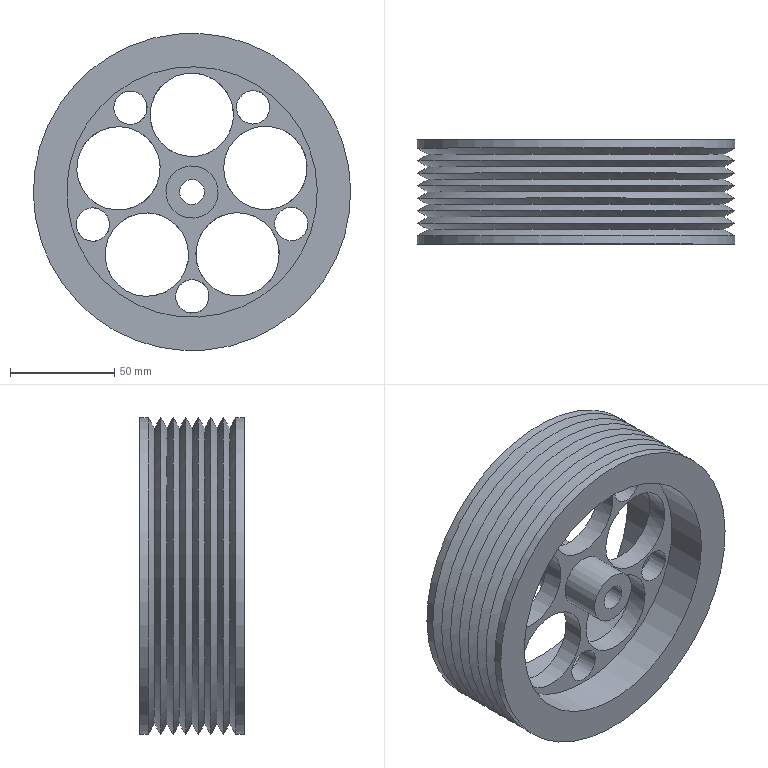Component | NX | LARGE_PULLEY | 1 solid | 37 faces | volume 345078 mm3 | cylinder 17 | cone 14 | plane 6 | commonest cylinder face diameters 16 x5 40 x5 152 x2 120 x2 25 x2 12 x1